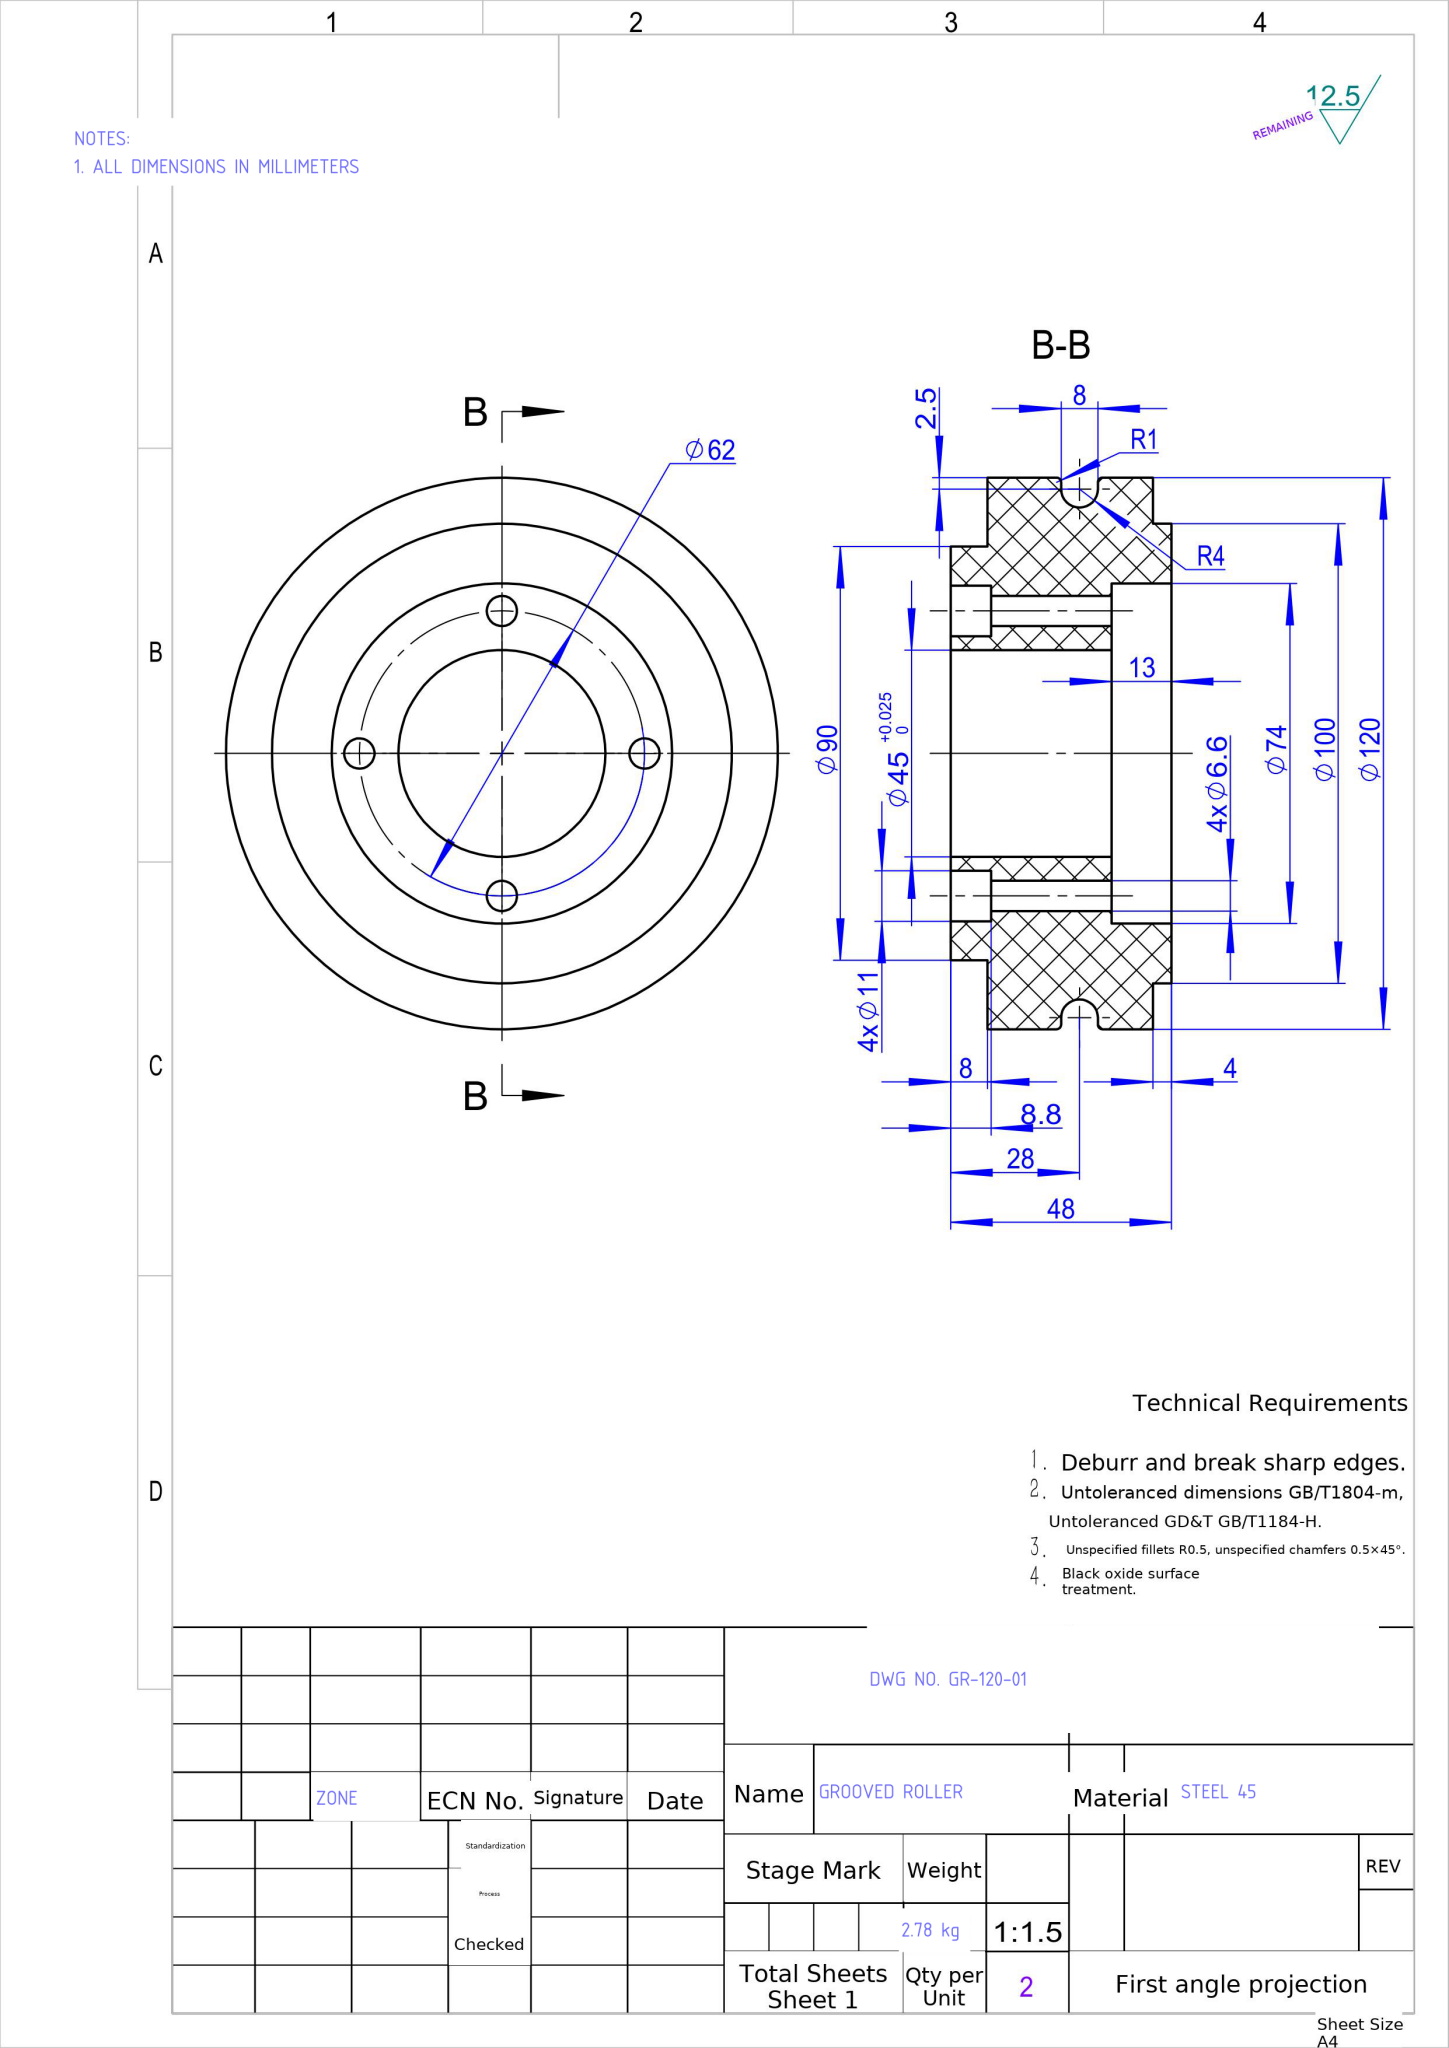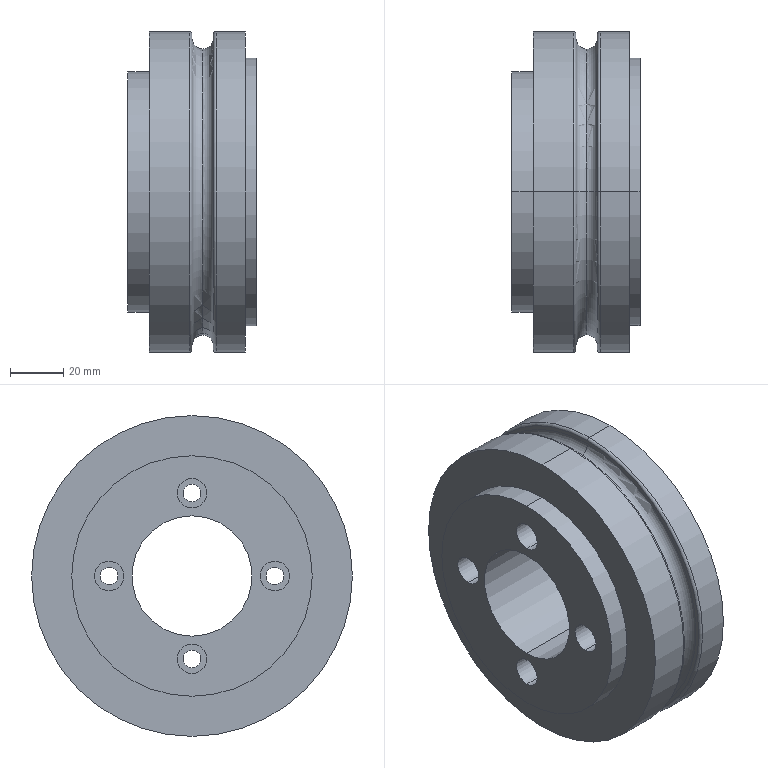Part | NX | mm | 1 solid | 47 faces | box 48 x 120 x 120 mm | volume 354598 mm3 | cylinder 28 | plane 11 | torus 8 | commonest cylinder face diameters 11 x8 6.6 x8 120 x4 100 x2 74 x2 45 x2 90 x2